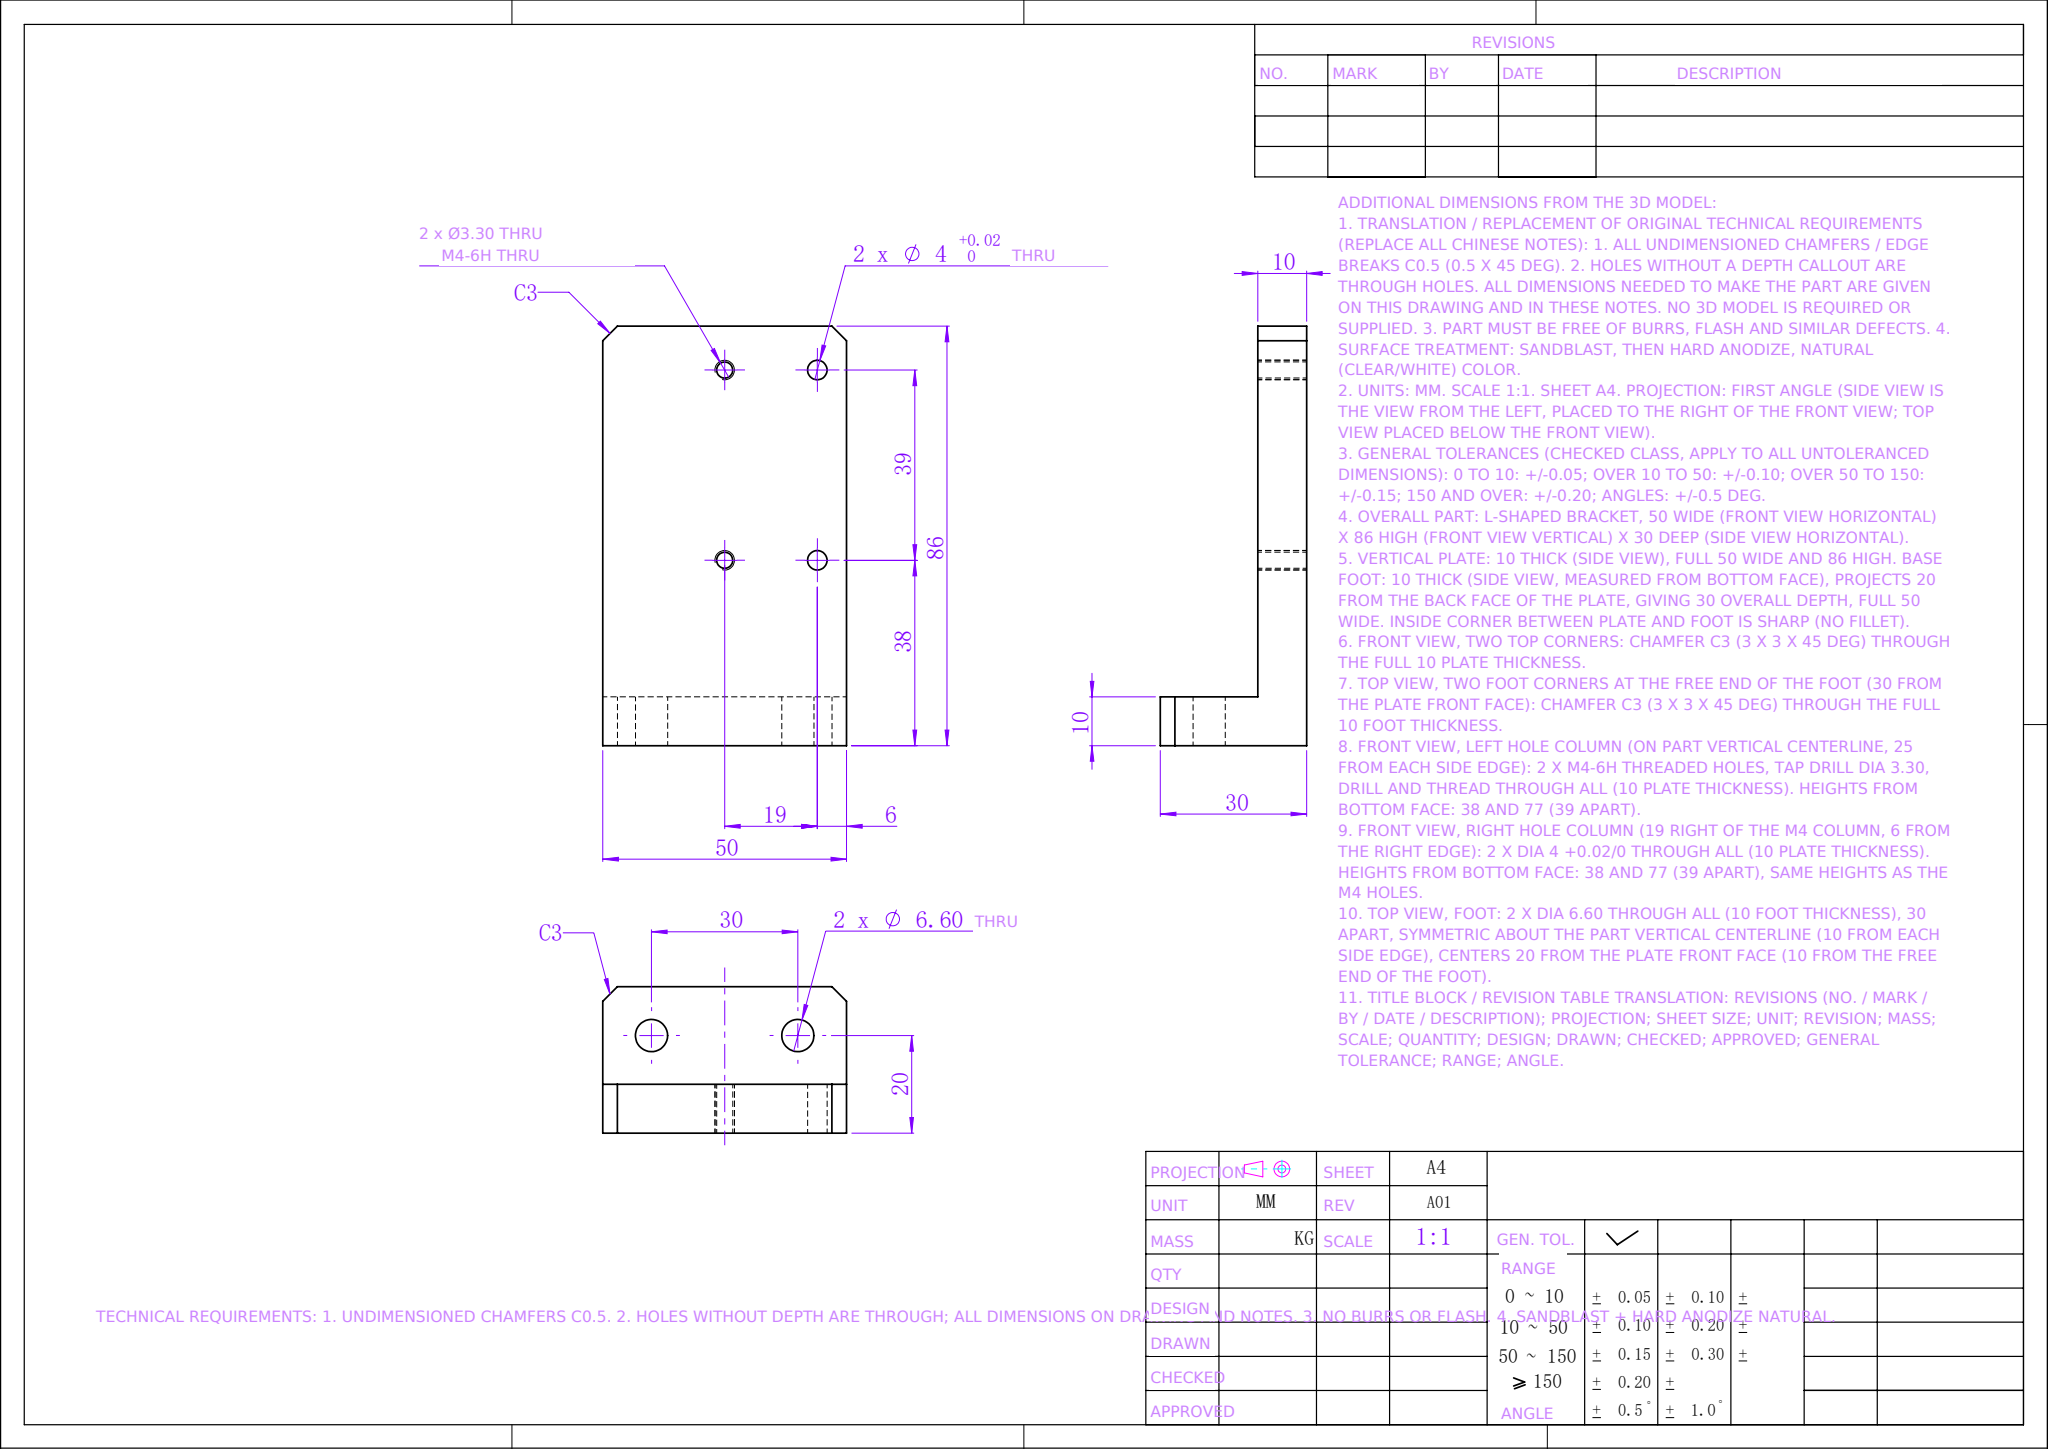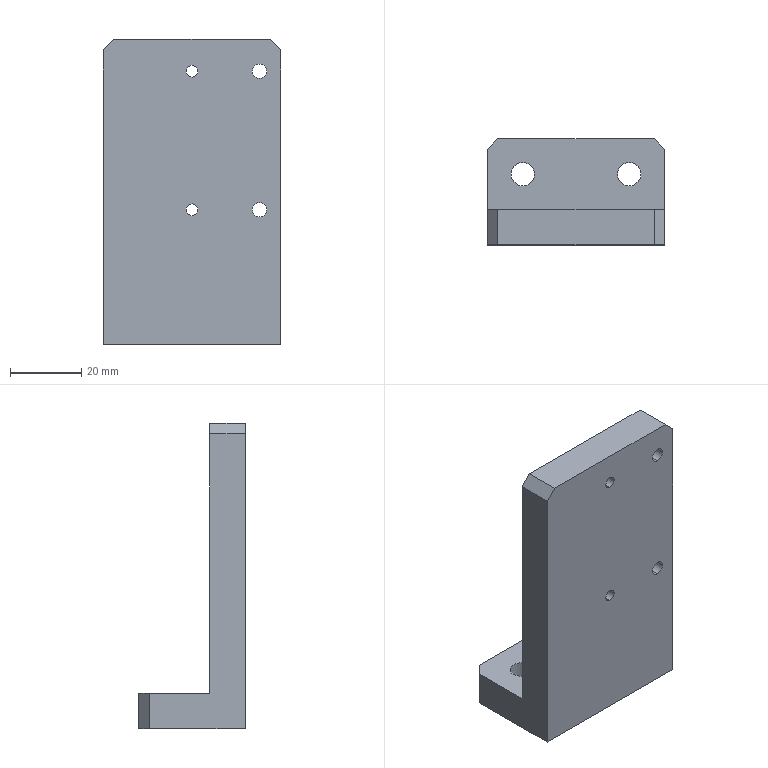Part | NX | mm | 1 solid | 24 faces | box 50 x 30 x 86 mm | volume 51713 mm3 | cylinder 12 | plane 12 | commonest cylinder face diameters 6.6 x4 4 x4 3.3 x4
STEP:
#1=COLOUR_RGB('',0.7922,0.8196,0.9333);
#2=FILL_AREA_STYLE_COLOUR('',#1);
#3=FILL_AREA_STYLE('',(#2));
#4=SURFACE_STYLE_FILL_AREA(#3);
#5=SURFACE_SIDE_STYLE('',(#4));
#6=SURFACE_STYLE_USAGE(.BOTH.,#5);
#7=PRESENTATION_STYLE_ASSIGNMENT((#6));
#8=CARTESIAN_POINT('',(-18.3,15.,-43.));
#9=VERTEX_POINT('',#8);
#10=CARTESIAN_POINT('',(-11.7,15.,-43.));
#11=VERTEX_POINT('',#10);
#12=CARTESIAN_POINT('',(-15.,15.,-43.));
#13=DIRECTION('',(0.,0.,1.));
#14=DIRECTION('',(1.,0.,0.));
#15=AXIS2_PLACEMENT_3D('',#12,#13,#14);
#16=CIRCLE('',#15,3.3);
#17=EDGE_CURVE('',#9,#11,#16,.T.);
#18=ORIENTED_EDGE('',*,*,#17,.F.);
#19=CARTESIAN_POINT('',(-18.3,15.,-33.));
#20=VERTEX_POINT('',#19);
#21=CARTESIAN_POINT('',(-18.3,15.,-33.));
#22=DIRECTION('',(0.,0.,1.));
#23=VECTOR('',#22,1000.);
#24=LINE('',#21,#23);
#25=EDGE_CURVE('',#9,#20,#24,.T.);
#26=ORIENTED_EDGE('',*,*,#25,.T.);
#27=CARTESIAN_POINT('',(-11.7,15.,-33.));
#28=VERTEX_POINT('',#27);
#29=CARTESIAN_POINT('',(-15.,15.,-33.));
#30=DIRECTION('',(0.,0.,1.));
#31=DIRECTION('',(1.,0.,0.));
#32=AXIS2_PLACEMENT_3D('',#29,#30,#31);
#33=CIRCLE('',#32,3.3);
#34=EDGE_CURVE('',#20,#28,#33,.T.);
#35=ORIENTED_EDGE('',*,*,#34,.T.);
#36=CARTESIAN_POINT('',(-11.7,15.,-33.));
#37=DIRECTION('',(0.,0.,1.));
#38=VECTOR('',#37,1000.);
#39=LINE('',#36,#38);
#40=EDGE_CURVE('',#11,#28,#39,.T.);
#41=ORIENTED_EDGE('',*,*,#40,.F.);
#42=EDGE_LOOP('',(#18,#26,#35,#41));
#43=FACE_OUTER_BOUND('',#42,.T.);
#44=CARTESIAN_POINT('',(-15.,15.,-33.));
#45=DIRECTION('',(0.,0.,1.));
#46=DIRECTION('',(1.,0.,0.));
#47=AXIS2_PLACEMENT_3D('',#44,#45,#46);
#48=CYLINDRICAL_SURFACE('',#47,3.3);
#49=ADVANCED_FACE('',(#43),#48,.F.);
#50=CARTESIAN_POINT('',(11.7,15.,-43.));
#51=VERTEX_POINT('',#50);
#52=CARTESIAN_POINT('',(18.3,15.,-43.));
#53=VERTEX_POINT('',#52);
#54=CARTESIAN_POINT('',(15.,15.,-43.));
#55=DIRECTION('',(0.,0.,1.));
#56=DIRECTION('',(1.,0.,0.));
#57=AXIS2_PLACEMENT_3D('',#54,#55,#56);
#58=CIRCLE('',#57,3.3);
#59=EDGE_CURVE('',#51,#53,#58,.T.);
#60=ORIENTED_EDGE('',*,*,#59,.F.);
#61=CARTESIAN_POINT('',(11.7,15.,-33.));
#62=VERTEX_POINT('',#61);
#63=CARTESIAN_POINT('',(11.7,15.,-33.));
#64=DIRECTION('',(0.,0.,1.));
#65=VECTOR('',#64,1000.);
#66=LINE('',#63,#65);
#67=EDGE_CURVE('',#51,#62,#66,.T.);
#68=ORIENTED_EDGE('',*,*,#67,.T.);
#69=CARTESIAN_POINT('',(18.3,15.,-33.));
#70=VERTEX_POINT('',#69);
#71=CARTESIAN_POINT('',(15.,15.,-33.));
#72=DIRECTION('',(0.,0.,1.));
#73=DIRECTION('',(1.,0.,0.));
#74=AXIS2_PLACEMENT_3D('',#71,#72,#73);
#75=CIRCLE('',#74,3.3);
#76=EDGE_CURVE('',#62,#70,#75,.T.);
#77=ORIENTED_EDGE('',*,*,#76,.T.);
#78=CARTESIAN_POINT('',(18.3,15.,-33.));
#79=DIRECTION('',(0.,0.,1.));
#80=VECTOR('',#79,1000.);
#81=LINE('',#78,#80);
#82=EDGE_CURVE('',#53,#70,#81,.T.);
#83=ORIENTED_EDGE('',*,*,#82,.F.);
#84=EDGE_LOOP('',(#60,#68,#77,#83));
#85=FACE_OUTER_BOUND('',#84,.T.);
#86=CARTESIAN_POINT('',(15.,15.,-33.));
#87=DIRECTION('',(0.,0.,1.));
#88=DIRECTION('',(1.,0.,0.));
#89=AXIS2_PLACEMENT_3D('',#86,#87,#88);
#90=CYLINDRICAL_SURFACE('',#89,3.3);
#91=ADVANCED_FACE('',(#85),#90,.F.);
#92=CARTESIAN_POINT('',(19.,-5.,32.));
#93=VERTEX_POINT('',#92);
#94=CARTESIAN_POINT('',(19.,-5.,36.));
#95=VERTEX_POINT('',#94);
#96=CARTESIAN_POINT('',(19.,-5.,34.));
#97=DIRECTION('',(0.,1.,0.));
#98=DIRECTION('',(0.,0.,1.));
#99=AXIS2_PLACEMENT_3D('',#96,#97,#98);
#100=CIRCLE('',#99,2.);
#101=EDGE_CURVE('',#93,#95,#100,.T.);
#102=ORIENTED_EDGE('',*,*,#101,.F.);
#103=CARTESIAN_POINT('',(19.,5.,32.));
#104=VERTEX_POINT('',#103);
#105=CARTESIAN_POINT('',(19.,5.,32.));
#106=DIRECTION('',(0.,1.,0.));
#107=VECTOR('',#106,1000.);
#108=LINE('',#105,#107);
#109=EDGE_CURVE('',#93,#104,#108,.T.);
#110=ORIENTED_EDGE('',*,*,#109,.T.);
#111=CARTESIAN_POINT('',(19.,5.,36.));
#112=VERTEX_POINT('',#111);
#113=CARTESIAN_POINT('',(19.,5.,34.));
#114=DIRECTION('',(0.,1.,0.));
#115=DIRECTION('',(0.,0.,1.));
#116=AXIS2_PLACEMENT_3D('',#113,#114,#115);
#117=CIRCLE('',#116,2.);
#118=EDGE_CURVE('',#104,#112,#117,.T.);
#119=ORIENTED_EDGE('',*,*,#118,.T.);
#120=CARTESIAN_POINT('',(19.,5.,36.));
#121=DIRECTION('',(0.,1.,0.));
#122=VECTOR('',#121,1000.);
#123=LINE('',#120,#122);
#124=EDGE_CURVE('',#95,#112,#123,.T.);
#125=ORIENTED_EDGE('',*,*,#124,.F.);
#126=EDGE_LOOP('',(#102,#110,#119,#125));
#127=FACE_OUTER_BOUND('',#126,.T.);
#128=CARTESIAN_POINT('',(19.,5.,34.));
#129=DIRECTION('',(0.,1.,0.));
#130=DIRECTION('',(0.,0.,1.));
#131=AXIS2_PLACEMENT_3D('',#128,#129,#130);
#132=CYLINDRICAL_SURFACE('',#131,2.);
#133=ADVANCED_FACE('',(#127),#132,.F.);
#134=CARTESIAN_POINT('',(19.,-5.,-7.));
#135=VERTEX_POINT('',#134);
#136=CARTESIAN_POINT('',(19.,-5.,-3.));
#137=VERTEX_POINT('',#136);
#138=CARTESIAN_POINT('',(19.,-5.,-5.));
#139=DIRECTION('',(0.,1.,0.));
#140=DIRECTION('',(0.,0.,1.));
#141=AXIS2_PLACEMENT_3D('',#138,#139,#140);
#142=CIRCLE('',#141,2.);
#143=EDGE_CURVE('',#135,#137,#142,.T.);
#144=ORIENTED_EDGE('',*,*,#143,.F.);
#145=CARTESIAN_POINT('',(19.,5.,-7.));
#146=VERTEX_POINT('',#145);
#147=CARTESIAN_POINT('',(19.,5.,-7.));
#148=DIRECTION('',(0.,1.,0.));
#149=VECTOR('',#148,1000.);
#150=LINE('',#147,#149);
#151=EDGE_CURVE('',#135,#146,#150,.T.);
#152=ORIENTED_EDGE('',*,*,#151,.T.);
#153=CARTESIAN_POINT('',(19.,5.,-3.));
#154=VERTEX_POINT('',#153);
#155=CARTESIAN_POINT('',(19.,5.,-5.));
#156=DIRECTION('',(0.,1.,0.));
#157=DIRECTION('',(0.,0.,1.));
#158=AXIS2_PLACEMENT_3D('',#155,#156,#157);
#159=CIRCLE('',#158,2.);
#160=EDGE_CURVE('',#146,#154,#159,.T.);
#161=ORIENTED_EDGE('',*,*,#160,.T.);
#162=CARTESIAN_POINT('',(19.,5.,-3.));
#163=DIRECTION('',(0.,1.,0.));
#164=VECTOR('',#163,1000.);
#165=LINE('',#162,#164);
#166=EDGE_CURVE('',#137,#154,#165,.T.);
#167=ORIENTED_EDGE('',*,*,#166,.F.);
#168=EDGE_LOOP('',(#144,#152,#161,#167));
#169=FACE_OUTER_BOUND('',#168,.T.);
#170=CARTESIAN_POINT('',(19.,5.,-5.));
#171=DIRECTION('',(0.,1.,0.));
#172=DIRECTION('',(0.,0.,1.));
#173=AXIS2_PLACEMENT_3D('',#170,#171,#172);
#174=CYLINDRICAL_SURFACE('',#173,2.);
#175=ADVANCED_FACE('',(#169),#174,.F.);
#176=CARTESIAN_POINT('',(-0.,5.,35.65));
#177=VERTEX_POINT('',#176);
#178=CARTESIAN_POINT('',(-0.,5.,32.35));
#179=VERTEX_POINT('',#178);
#180=CARTESIAN_POINT('',(-0.,5.,34.));
#181=DIRECTION('',(0.,-1.,0.));
#182=DIRECTION('',(0.,0.,-1.));
#183=AXIS2_PLACEMENT_3D('',#180,#181,#182);
#184=CIRCLE('',#183,1.65);
#185=EDGE_CURVE('',#177,#179,#184,.T.);
#186=ORIENTED_EDGE('',*,*,#185,.F.);
#187=CARTESIAN_POINT('',(-0.,-5.,35.65));
#188=VERTEX_POINT('',#187);
#189=CARTESIAN_POINT('',(-0.,-5.,35.65));
#190=DIRECTION('',(0.,-1.,0.));
#191=VECTOR('',#190,1000.);
#192=LINE('',#189,#191);
#193=EDGE_CURVE('',#177,#188,#192,.T.);
#194=ORIENTED_EDGE('',*,*,#193,.T.);
#195=CARTESIAN_POINT('',(-0.,-5.,32.35));
#196=VERTEX_POINT('',#195);
#197=CARTESIAN_POINT('',(-0.,-5.,34.));
#198=DIRECTION('',(0.,-1.,0.));
#199=DIRECTION('',(0.,0.,-1.));
#200=AXIS2_PLACEMENT_3D('',#197,#198,#199);
#201=CIRCLE('',#200,1.65);
#202=EDGE_CURVE('',#188,#196,#201,.T.);
#203=ORIENTED_EDGE('',*,*,#202,.T.);
#204=CARTESIAN_POINT('',(-0.,-5.,32.35));
#205=DIRECTION('',(0.,-1.,0.));
#206=VECTOR('',#205,1000.);
#207=LINE('',#204,#206);
#208=EDGE_CURVE('',#179,#196,#207,.T.);
#209=ORIENTED_EDGE('',*,*,#208,.F.);
#210=EDGE_LOOP('',(#186,#194,#203,#209));
#211=FACE_OUTER_BOUND('',#210,.T.);
#212=CARTESIAN_POINT('',(-0.,-5.,34.));
#213=DIRECTION('',(0.,-1.,0.));
#214=DIRECTION('',(0.,0.,-1.));
#215=AXIS2_PLACEMENT_3D('',#212,#213,#214);
#216=CYLINDRICAL_SURFACE('',#215,1.65);
#217=ADVANCED_FACE('',(#211),#216,.F.);
#218=CARTESIAN_POINT('',(0.,5.,-3.35));
#219=VERTEX_POINT('',#218);
#220=CARTESIAN_POINT('',(0.,5.,-6.65));
#221=VERTEX_POINT('',#220);
#222=CARTESIAN_POINT('',(0.,5.,-5.));
#223=DIRECTION('',(0.,-1.,0.));
#224=DIRECTION('',(0.,0.,-1.));
#225=AXIS2_PLACEMENT_3D('',#222,#223,#224);
#226=CIRCLE('',#225,1.65);
#227=EDGE_CURVE('',#219,#221,#226,.T.);
#228=ORIENTED_EDGE('',*,*,#227,.F.);
#229=CARTESIAN_POINT('',(0.,-5.,-3.35));
#230=VERTEX_POINT('',#229);
#231=CARTESIAN_POINT('',(0.,-5.,-3.35));
#232=DIRECTION('',(0.,-1.,0.));
#233=VECTOR('',#232,1000.);
#234=LINE('',#231,#233);
#235=EDGE_CURVE('',#219,#230,#234,.T.);
#236=ORIENTED_EDGE('',*,*,#235,.T.);
#237=CARTESIAN_POINT('',(0.,-5.,-6.65));
#238=VERTEX_POINT('',#237);
#239=CARTESIAN_POINT('',(0.,-5.,-5.));
#240=DIRECTION('',(0.,-1.,0.));
#241=DIRECTION('',(0.,0.,-1.));
#242=AXIS2_PLACEMENT_3D('',#239,#240,#241);
#243=CIRCLE('',#242,1.65);
#244=EDGE_CURVE('',#230,#238,#243,.T.);
#245=ORIENTED_EDGE('',*,*,#244,.T.);
#246=CARTESIAN_POINT('',(0.,-5.,-6.65));
#247=DIRECTION('',(0.,-1.,0.));
#248=VECTOR('',#247,1000.);
#249=LINE('',#246,#248);
#250=EDGE_CURVE('',#221,#238,#249,.T.);
#251=ORIENTED_EDGE('',*,*,#250,.F.);
#252=EDGE_LOOP('',(#228,#236,#245,#251));
#253=FACE_OUTER_BOUND('',#252,.T.);
#254=CARTESIAN_POINT('',(0.,-5.,-5.));
#255=DIRECTION('',(0.,-1.,0.));
#256=DIRECTION('',(0.,0.,-1.));
#257=AXIS2_PLACEMENT_3D('',#254,#255,#256);
#258=CYLINDRICAL_SURFACE('',#257,1.65);
#259=ADVANCED_FACE('',(#253),#258,.F.);
#260=CARTESIAN_POINT('',(19.,5.,-5.));
#261=DIRECTION('',(0.,1.,0.));
#262=DIRECTION('',(0.,0.,1.));
#263=AXIS2_PLACEMENT_3D('',#260,#261,#262);
#264=CIRCLE('',#263,2.);
#265=EDGE_CURVE('',#154,#146,#264,.T.);
#266=ORIENTED_EDGE('',*,*,#265,.F.);
#267=ORIENTED_EDGE('',*,*,#160,.F.);
#268=EDGE_LOOP('',(#266,#267));
#269=FACE_BOUND('',#268,.T.);
#270=CARTESIAN_POINT('',(-0.,5.,34.));
#271=DIRECTION('',(0.,-1.,0.));
#272=DIRECTION('',(0.,0.,-1.));
#273=AXIS2_PLACEMENT_3D('',#270,#271,#272);
#274=CIRCLE('',#273,1.65);
#275=EDGE_CURVE('',#179,#177,#274,.T.);
#276=ORIENTED_EDGE('',*,*,#275,.T.);
#277=ORIENTED_EDGE('',*,*,#185,.T.);
#278=EDGE_LOOP('',(#276,#277));
#279=FACE_BOUND('',#278,.T.);
#280=CARTESIAN_POINT('',(0.,5.,-5.));
#281=DIRECTION('',(0.,-1.,0.));
#282=DIRECTION('',(0.,0.,-1.));
#283=AXIS2_PLACEMENT_3D('',#280,#281,#282);
#284=CIRCLE('',#283,1.65);
#285=EDGE_CURVE('',#221,#219,#284,.T.);
#286=ORIENTED_EDGE('',*,*,#285,.T.);
#287=ORIENTED_EDGE('',*,*,#227,.T.);
#288=EDGE_LOOP('',(#286,#287));
#289=FACE_BOUND('',#288,.T.);
#290=CARTESIAN_POINT('',(-25.,5.,40.));
#291=VERTEX_POINT('',#290);
#292=CARTESIAN_POINT('',(-25.,5.,-33.));
#293=VERTEX_POINT('',#292);
#294=CARTESIAN_POINT('',(-25.,5.,43.));
#295=DIRECTION('',(0.,0.,-1.));
#296=VECTOR('',#295,1000.);
#297=LINE('',#294,#296);
#298=EDGE_CURVE('',#291,#293,#297,.T.);
#299=ORIENTED_EDGE('',*,*,#298,.F.);
#300=CARTESIAN_POINT('',(-22.,5.,43.));
#301=VERTEX_POINT('',#300);
#302=CARTESIAN_POINT('',(-22.,5.,43.));
#303=DIRECTION('',(0.7071,0.,0.7071));
#304=VECTOR('',#303,1000.);
#305=LINE('',#302,#304);
#306=EDGE_CURVE('',#291,#301,#305,.T.);
#307=ORIENTED_EDGE('',*,*,#306,.T.);
#308=CARTESIAN_POINT('',(22.,5.,43.));
#309=VERTEX_POINT('',#308);
#310=CARTESIAN_POINT('',(-25.,5.,43.));
#311=DIRECTION('',(-1.,0.,0.));
#312=VECTOR('',#311,1000.);
#313=LINE('',#310,#312);
#314=EDGE_CURVE('',#309,#301,#313,.T.);
#315=ORIENTED_EDGE('',*,*,#314,.F.);
#316=CARTESIAN_POINT('',(25.,5.,40.));
#317=VERTEX_POINT('',#316);
#318=CARTESIAN_POINT('',(22.,5.,43.));
#319=DIRECTION('',(0.7071,0.,-0.7071));
#320=VECTOR('',#319,1000.);
#321=LINE('',#318,#320);
#322=EDGE_CURVE('',#309,#317,#321,.T.);
#323=ORIENTED_EDGE('',*,*,#322,.T.);
#324=CARTESIAN_POINT('',(25.,5.,-33.));
#325=VERTEX_POINT('',#324);
#326=CARTESIAN_POINT('',(25.,5.,43.));
#327=DIRECTION('',(0.,0.,-1.));
#328=VECTOR('',#327,1000.);
#329=LINE('',#326,#328);
#330=EDGE_CURVE('',#317,#325,#329,.T.);
#331=ORIENTED_EDGE('',*,*,#330,.T.);
#332=CARTESIAN_POINT('',(25.,5.,-33.));
#333=DIRECTION('',(1.,0.,-0.));
#334=VECTOR('',#333,1000.);
#335=LINE('',#332,#334);
#336=EDGE_CURVE('',#293,#325,#335,.T.);
#337=ORIENTED_EDGE('',*,*,#336,.F.);
#338=EDGE_LOOP('',(#299,#307,#315,#323,#331,#337));
#339=FACE_OUTER_BOUND('',#338,.T.);
#340=CARTESIAN_POINT('',(19.,5.,34.));
#341=DIRECTION('',(0.,1.,0.));
#342=DIRECTION('',(0.,0.,1.));
#343=AXIS2_PLACEMENT_3D('',#340,#341,#342);
#344=CIRCLE('',#343,2.);
#345=EDGE_CURVE('',#112,#104,#344,.T.);
#346=ORIENTED_EDGE('',*,*,#345,.F.);
#347=ORIENTED_EDGE('',*,*,#118,.F.);
#348=EDGE_LOOP('',(#346,#347));
#349=FACE_BOUND('',#348,.T.);
#350=CARTESIAN_POINT('',(-25.,5.,43.));
#351=DIRECTION('',(0.,-1.,0.));
#352=DIRECTION('',(0.,0.,-1.));
#353=AXIS2_PLACEMENT_3D('',#350,#351,#352);
#354=PLANE('',#353);
#355=ADVANCED_FACE('',(#269,#279,#289,#339,#349),#354,.F.);
#356=CARTESIAN_POINT('',(25.,-5.,-43.));
#357=VERTEX_POINT('',#356);
#358=CARTESIAN_POINT('',(25.,22.,-43.));
#359=VERTEX_POINT('',#358);
#360=CARTESIAN_POINT('',(25.,-5.,-43.));
#361=DIRECTION('',(0.,1.,0.));
#362=VECTOR('',#361,1000.);
#363=LINE('',#360,#362);
#364=EDGE_CURVE('',#357,#359,#363,.T.);
#365=ORIENTED_EDGE('',*,*,#364,.T.);
#366=CARTESIAN_POINT('',(25.,22.,-33.));
#367=VERTEX_POINT('',#366);
#368=CARTESIAN_POINT('',(25.,22.,43.));
#369=DIRECTION('',(0.,0.,1.));
#370=VECTOR('',#369,1000.);
#371=LINE('',#368,#370);
#372=EDGE_CURVE('',#359,#367,#371,.T.);
#373=ORIENTED_EDGE('',*,*,#372,.T.);
#374=CARTESIAN_POINT('',(25.,25.,-33.));
#375=DIRECTION('',(0.,-1.,0.));
#376=VECTOR('',#375,1000.);
#377=LINE('',#374,#376);
#378=EDGE_CURVE('',#367,#325,#377,.T.);
#379=ORIENTED_EDGE('',*,*,#378,.T.);
#380=ORIENTED_EDGE('',*,*,#330,.F.);
#381=CARTESIAN_POINT('',(25.,-5.,40.));
#382=VERTEX_POINT('',#381);
#383=CARTESIAN_POINT('',(25.,-5.,40.));
#384=DIRECTION('',(0.,-1.,0.));
#385=VECTOR('',#384,1000.);
#386=LINE('',#383,#385);
#387=EDGE_CURVE('',#317,#382,#386,.T.);
#388=ORIENTED_EDGE('',*,*,#387,.T.);
#389=CARTESIAN_POINT('',(25.,-5.,43.));
#390=DIRECTION('',(0.,0.,-1.));
#391=VECTOR('',#390,1000.);
#392=LINE('',#389,#391);
#393=EDGE_CURVE('',#382,#357,#392,.T.);
#394=ORIENTED_EDGE('',*,*,#393,.T.);
#395=EDGE_LOOP('',(#365,#373,#379,#380,#388,#394));
#396=FACE_OUTER_BOUND('',#395,.T.);
#397=CARTESIAN_POINT('',(25.,-5.,43.));
#398=DIRECTION('',(-1.,0.,0.));
#399=DIRECTION('',(0.,0.,1.));
#400=AXIS2_PLACEMENT_3D('',#397,#398,#399);
#401=PLANE('',#400);
#402=ADVANCED_FACE('',(#396),#401,.F.);
#403=CARTESIAN_POINT('',(-25.,22.,-33.));
#404=VERTEX_POINT('',#403);
#405=CARTESIAN_POINT('',(-25.,25.,-33.));
#406=DIRECTION('',(0.,-1.,0.));
#407=VECTOR('',#406,1000.);
#408=LINE('',#405,#407);
#409=EDGE_CURVE('',#404,#293,#408,.T.);
#410=ORIENTED_EDGE('',*,*,#409,.F.);
#411=CARTESIAN_POINT('',(-25.,22.,-43.));
#412=VERTEX_POINT('',#411);
#413=CARTESIAN_POINT('',(-25.,22.,43.));
#414=DIRECTION('',(0.,0.,-1.));
#415=VECTOR('',#414,1000.);
#416=LINE('',#413,#415);
#417=EDGE_CURVE('',#404,#412,#416,.T.);
#418=ORIENTED_EDGE('',*,*,#417,.T.);
#419=CARTESIAN_POINT('',(-25.,-5.,-43.));
#420=VERTEX_POINT('',#419);
#421=CARTESIAN_POINT('',(-25.,-5.,-43.));
#422=DIRECTION('',(0.,-1.,0.));
#423=VECTOR('',#422,1000.);
#424=LINE('',#421,#423);
#425=EDGE_CURVE('',#412,#420,#424,.T.);
#426=ORIENTED_EDGE('',*,*,#425,.T.);
#427=CARTESIAN_POINT('',(-25.,-5.,40.));
#428=VERTEX_POINT('',#427);
#429=CARTESIAN_POINT('',(-25.,-5.,43.));
#430=DIRECTION('',(0.,0.,-1.));
#431=VECTOR('',#430,1000.);
#432=LINE('',#429,#431);
#433=EDGE_CURVE('',#428,#420,#432,.T.);
#434=ORIENTED_EDGE('',*,*,#433,.F.);
#435=CARTESIAN_POINT('',(-25.,-5.,40.));
#436=DIRECTION('',(0.,1.,0.));
#437=VECTOR('',#436,1000.);
#438=LINE('',#435,#437);
#439=EDGE_CURVE('',#428,#291,#438,.T.);
#440=ORIENTED_EDGE('',*,*,#439,.T.);
#441=ORIENTED_EDGE('',*,*,#298,.T.);
#442=EDGE_LOOP('',(#410,#418,#426,#434,#440,#441));
#443=FACE_OUTER_BOUND('',#442,.T.);
#444=CARTESIAN_POINT('',(-25.,-5.,43.));
#445=DIRECTION('',(1.,0.,0.));
#446=DIRECTION('',(0.,0.,-1.));
#447=AXIS2_PLACEMENT_3D('',#444,#445,#446);
#448=PLANE('',#447);
#449=ADVANCED_FACE('',(#443),#448,.F.);
#450=CARTESIAN_POINT('',(19.,-5.,34.));
#451=DIRECTION('',(0.,1.,0.));
#452=DIRECTION('',(0.,0.,1.));
#453=AXIS2_PLACEMENT_3D('',#450,#451,#452);
#454=CIRCLE('',#453,2.);
#455=EDGE_CURVE('',#95,#93,#454,.T.);
#456=ORIENTED_EDGE('',*,*,#455,.T.);
#457=ORIENTED_EDGE('',*,*,#101,.T.);
#458=EDGE_LOOP('',(#456,#457));
#459=FACE_BOUND('',#458,.T.);
#460=CARTESIAN_POINT('',(19.,-5.,-5.));
#461=DIRECTION('',(0.,1.,0.));
#462=DIRECTION('',(0.,0.,1.));
#463=AXIS2_PLACEMENT_3D('',#460,#461,#462);
#464=CIRCLE('',#463,2.);
#465=EDGE_CURVE('',#137,#135,#464,.T.);
#466=ORIENTED_EDGE('',*,*,#465,.T.);
#467=ORIENTED_EDGE('',*,*,#143,.T.);
#468=EDGE_LOOP('',(#466,#467));
#469=FACE_BOUND('',#468,.T.);
#470=CARTESIAN_POINT('',(-0.,-5.,34.));
#471=DIRECTION('',(0.,-1.,0.));
#472=DIRECTION('',(0.,0.,-1.));
#473=AXIS2_PLACEMENT_3D('',#470,#471,#472);
#474=CIRCLE('',#473,1.65);
#475=EDGE_CURVE('',#196,#188,#474,.T.);
#476=ORIENTED_EDGE('',*,*,#475,.F.);
#477=ORIENTED_EDGE('',*,*,#202,.F.);
#478=EDGE_LOOP('',(#476,#477));
#479=FACE_BOUND('',#478,.T.);
#480=CARTESIAN_POINT('',(0.,-5.,-5.));
#481=DIRECTION('',(0.,-1.,0.));
#482=DIRECTION('',(0.,0.,-1.));
#483=AXIS2_PLACEMENT_3D('',#480,#481,#482);
#484=CIRCLE('',#483,1.65);
#485=EDGE_CURVE('',#238,#230,#484,.T.);
#486=ORIENTED_EDGE('',*,*,#485,.F.);
#487=ORIENTED_EDGE('',*,*,#244,.F.);
#488=EDGE_LOOP('',(#486,#487));
#489=FACE_BOUND('',#488,.T.);
#490=CARTESIAN_POINT('',(-22.,-5.,43.));
#491=VERTEX_POINT('',#490);
#492=CARTESIAN_POINT('',(22.,-5.,43.));
#493=VERTEX_POINT('',#492);
#494=CARTESIAN_POINT('',(-25.,-5.,43.));
#495=DIRECTION('',(1.,0.,0.));
#496=VECTOR('',#495,1000.);
#497=LINE('',#494,#496);
#498=EDGE_CURVE('',#491,#493,#497,.T.);
#499=ORIENTED_EDGE('',*,*,#498,.F.);
#500=CARTESIAN_POINT('',(-22.,-5.,43.));
#501=DIRECTION('',(-0.7071,0.,-0.7071));
#502=VECTOR('',#501,1000.);
#503=LINE('',#500,#502);
#504=EDGE_CURVE('',#491,#428,#503,.T.);
#505=ORIENTED_EDGE('',*,*,#504,.T.);
#506=ORIENTED_EDGE('',*,*,#433,.T.);
#507=CARTESIAN_POINT('',(-25.,-5.,-43.));
#508=DIRECTION('',(1.,0.,0.));
#509=VECTOR('',#508,1000.);
#510=LINE('',#507,#509);
#511=EDGE_CURVE('',#420,#357,#510,.T.);
#512=ORIENTED_EDGE('',*,*,#511,.T.);
#513=ORIENTED_EDGE('',*,*,#393,.F.);
#514=CARTESIAN_POINT('',(22.,-5.,43.));
#515=DIRECTION('',(-0.7071,0.,0.7071));
#516=VECTOR('',#515,1000.);
#517=LINE('',#514,#516);
#518=EDGE_CURVE('',#382,#493,#517,.T.);
#519=ORIENTED_EDGE('',*,*,#518,.T.);
#520=EDGE_LOOP('',(#499,#505,#506,#512,#513,#519));
#521=FACE_OUTER_BOUND('',#520,.T.);
#522=CARTESIAN_POINT('',(-25.,-5.,43.));
#523=DIRECTION('',(0.,1.,0.));
#524=DIRECTION('',(0.,0.,1.));
#525=AXIS2_PLACEMENT_3D('',#522,#523,#524);
#526=PLANE('',#525);
#527=ADVANCED_FACE('',(#459,#469,#479,#489,#521),#526,.F.);
#528=ORIENTED_EDGE('',*,*,#314,.T.);
#529=CARTESIAN_POINT('',(-22.,0.,43.));
#530=DIRECTION('',(0.,-1.,0.));
#531=VECTOR('',#530,1000.);
#532=LINE('',#529,#531);
#533=EDGE_CURVE('',#301,#491,#532,.T.);
#534=ORIENTED_EDGE('',*,*,#533,.T.);
#535=ORIENTED_EDGE('',*,*,#498,.T.);
#536=CARTESIAN_POINT('',(22.,0.,43.));
#537=DIRECTION('',(0.,1.,0.));
#538=VECTOR('',#537,1000.);
#539=LINE('',#536,#538);
#540=EDGE_CURVE('',#493,#309,#539,.T.);
#541=ORIENTED_EDGE('',*,*,#540,.T.);
#542=EDGE_LOOP('',(#528,#534,#535,#541));
#543=FACE_OUTER_BOUND('',#542,.T.);
#544=CARTESIAN_POINT('',(0.,0.,43.));
#545=DIRECTION('',(0.,0.,-1.));
#546=DIRECTION('',(-1.,0.,0.));
#547=AXIS2_PLACEMENT_3D('',#544,#545,#546);
#548=PLANE('',#547);
#549=ADVANCED_FACE('',(#543),#548,.F.);
#550=CARTESIAN_POINT('',(-15.,15.,-43.));
#551=DIRECTION('',(0.,0.,1.));
#552=DIRECTION('',(1.,0.,0.));
#553=AXIS2_PLACEMENT_3D('',#550,#551,#552);
#554=CIRCLE('',#553,3.3);
#555=EDGE_CURVE('',#11,#9,#554,.T.);
#556=ORIENTED_EDGE('',*,*,#555,.T.);
#557=ORIENTED_EDGE('',*,*,#17,.T.);
#558=EDGE_LOOP('',(#556,#557));
#559=FACE_BOUND('',#558,.T.);
#560=CARTESIAN_POINT('',(15.,15.,-43.));
#561=DIRECTION('',(0.,0.,1.));
#562=DIRECTION('',(1.,0.,0.));
#563=AXIS2_PLACEMENT_3D('',#560,#561,#562);
#564=CIRCLE('',#563,3.3);
#565=EDGE_CURVE('',#53,#51,#564,.T.);
#566=ORIENTED_EDGE('',*,*,#565,.T.);
#567=ORIENTED_EDGE('',*,*,#59,.T.);
#568=EDGE_LOOP('',(#566,#567));
#569=FACE_BOUND('',#568,.T.);
#570=CARTESIAN_POINT('',(22.,25.,-43.));
#571=VERTEX_POINT('',#570);
#572=CARTESIAN_POINT('',(-22.,25.,-43.));
#573=VERTEX_POINT('',#572);
#574=CARTESIAN_POINT('',(25.,25.,-43.));
#575=DIRECTION('',(-1.,0.,0.));
#576=VECTOR('',#575,1000.);
#577=LINE('',#574,#576);
#578=EDGE_CURVE('',#571,#573,#577,.T.);
#579=ORIENTED_EDGE('',*,*,#578,.F.);
#580=CARTESIAN_POINT('',(23.5,23.5,-43.));
#581=DIRECTION('',(0.7071,-0.7071,0.));
#582=VECTOR('',#581,1000.);
#583=LINE('',#580,#582);
#584=EDGE_CURVE('',#571,#359,#583,.T.);
#585=ORIENTED_EDGE('',*,*,#584,.T.);
#586=ORIENTED_EDGE('',*,*,#364,.F.);
#587=ORIENTED_EDGE('',*,*,#511,.F.);
#588=ORIENTED_EDGE('',*,*,#425,.F.);
#589=CARTESIAN_POINT('',(-23.5,23.5,-43.));
#590=DIRECTION('',(0.7071,0.7071,0.));
#591=VECTOR('',#590,1000.);
#592=LINE('',#589,#591);
#593=EDGE_CURVE('',#412,#573,#592,.T.);
#594=ORIENTED_EDGE('',*,*,#593,.T.);
#595=EDGE_LOOP('',(#579,#585,#586,#587,#588,#594));
#596=FACE_OUTER_BOUND('',#595,.T.);
#597=CARTESIAN_POINT('',(0.,0.,-43.));
#598=DIRECTION('',(0.,0.,-1.));
#599=DIRECTION('',(-1.,0.,0.));
#600=AXIS2_PLACEMENT_3D('',#597,#598,#599);
#601=PLANE('',#600);
#602=ADVANCED_FACE('',(#559,#569,#596),#601,.T.);
#603=CARTESIAN_POINT('',(-15.,15.,-33.));
#604=DIRECTION('',(0.,0.,1.));
#605=DIRECTION('',(1.,0.,0.));
#606=AXIS2_PLACEMENT_3D('',#603,#604,#605);
#607=CIRCLE('',#606,3.3);
#608=EDGE_CURVE('',#28,#20,#607,.T.);
#609=ORIENTED_EDGE('',*,*,#608,.F.);
#610=ORIENTED_EDGE('',*,*,#34,.F.);
#611=EDGE_LOOP('',(#609,#610));
#612=FACE_BOUND('',#611,.T.);
#613=CARTESIAN_POINT('',(15.,15.,-33.));
#614=DIRECTION('',(0.,0.,1.));
#615=DIRECTION('',(1.,0.,0.));
#616=AXIS2_PLACEMENT_3D('',#613,#614,#615);
#617=CIRCLE('',#616,3.3);
#618=EDGE_CURVE('',#70,#62,#617,.T.);
#619=ORIENTED_EDGE('',*,*,#618,.F.);
#620=ORIENTED_EDGE('',*,*,#76,.F.);
#621=EDGE_LOOP('',(#619,#620));
#622=FACE_BOUND('',#621,.T.);
#623=ORIENTED_EDGE('',*,*,#378,.F.);
#624=CARTESIAN_POINT('',(22.,25.,-33.));
#625=VERTEX_POINT('',#624);
#626=CARTESIAN_POINT('',(22.,25.,-33.));
#627=DIRECTION('',(-0.7071,0.7071,0.));
#628=VECTOR('',#627,1000.);
#629=LINE('',#626,#628);
#630=EDGE_CURVE('',#367,#625,#629,.T.);
#631=ORIENTED_EDGE('',*,*,#630,.T.);
#632=CARTESIAN_POINT('',(-22.,25.,-33.));
#633=VERTEX_POINT('',#632);
#634=CARTESIAN_POINT('',(25.,25.,-33.));
#635=DIRECTION('',(1.,0.,-0.));
#636=VECTOR('',#635,1000.);
#637=LINE('',#634,#636);
#638=EDGE_CURVE('',#633,#625,#637,.T.);
#639=ORIENTED_EDGE('',*,*,#638,.F.);
#640=CARTESIAN_POINT('',(-22.,25.,-33.));
#641=DIRECTION('',(-0.7071,-0.7071,0.));
#642=VECTOR('',#641,1000.);
#643=LINE('',#640,#642);
#644=EDGE_CURVE('',#633,#404,#643,.T.);
#645=ORIENTED_EDGE('',*,*,#644,.T.);
#646=ORIENTED_EDGE('',*,*,#409,.T.);
#647=ORIENTED_EDGE('',*,*,#336,.T.);
#648=EDGE_LOOP('',(#623,#631,#639,#645,#646,#647));
#649=FACE_OUTER_BOUND('',#648,.T.);
#650=CARTESIAN_POINT('',(25.,25.,-33.));
#651=DIRECTION('',(-0.,0.,-1.));
#652=DIRECTION('',(-1.,0.,0.));
#653=AXIS2_PLACEMENT_3D('',#650,#651,#652);
#654=PLANE('',#653);
#655=ADVANCED_FACE('',(#612,#622,#649),#654,.F.);
#656=ORIENTED_EDGE('',*,*,#638,.T.);
#657=CARTESIAN_POINT('',(22.,25.,0.));
#658=DIRECTION('',(0.,0.,-1.));
#659=VECTOR('',#658,1000.);
#660=LINE('',#657,#659);
#661=EDGE_CURVE('',#625,#571,#660,.T.);
#662=ORIENTED_EDGE('',*,*,#661,.T.);
#663=ORIENTED_EDGE('',*,*,#578,.T.);
#664=CARTESIAN_POINT('',(-22.,25.,0.));
#665=DIRECTION('',(0.,0.,1.));
#666=VECTOR('',#665,1000.);
#667=LINE('',#664,#666);
#668=EDGE_CURVE('',#573,#633,#667,.T.);
#669=ORIENTED_EDGE('',*,*,#668,.T.);
#670=EDGE_LOOP('',(#656,#662,#663,#669));
#671=FACE_OUTER_BOUND('',#670,.T.);
#672=CARTESIAN_POINT('',(0.,25.,0.));
#673=DIRECTION('',(0.,-1.,0.));
#674=DIRECTION('',(0.,0.,-1.));
#675=AXIS2_PLACEMENT_3D('',#672,#673,#674);
#676=PLANE('',#675);
#677=ADVANCED_FACE('',(#671),#676,.F.);
#678=ORIENTED_EDGE('',*,*,#630,.F.);
#679=ORIENTED_EDGE('',*,*,#372,.F.);
#680=ORIENTED_EDGE('',*,*,#584,.F.);
#681=ORIENTED_EDGE('',*,*,#661,.F.);
#682=EDGE_LOOP('',(#678,#679,#680,#681));
#683=FACE_OUTER_BOUND('',#682,.T.);
#684=CARTESIAN_POINT('',(22.,25.,0.));
#685=DIRECTION('',(-0.7071,-0.7071,0.));
#686=DIRECTION('',(0.,0.,-1.));
#687=AXIS2_PLACEMENT_3D('',#684,#685,#686);
#688=PLANE('',#687);
#689=ADVANCED_FACE('',(#683),#688,.F.);
#690=ORIENTED_EDGE('',*,*,#593,.F.);
#691=ORIENTED_EDGE('',*,*,#417,.F.);
#692=ORIENTED_EDGE('',*,*,#644,.F.);
#693=ORIENTED_EDGE('',*,*,#668,.F.);
#694=EDGE_LOOP('',(#690,#691,#692,#693));
#695=FACE_OUTER_BOUND('',#694,.T.);
#696=CARTESIAN_POINT('',(-22.,25.,0.));
#697=DIRECTION('',(0.7071,-0.7071,0.));
#698=DIRECTION('',(0.,0.,1.));
#699=AXIS2_PLACEMENT_3D('',#696,#697,#698);
#700=PLANE('',#699);
#701=ADVANCED_FACE('',(#695),#700,.F.);
#702=ORIENTED_EDGE('',*,*,#306,.F.);
#703=ORIENTED_EDGE('',*,*,#439,.F.);
#704=ORIENTED_EDGE('',*,*,#504,.F.);
#705=ORIENTED_EDGE('',*,*,#533,.F.);
#706=EDGE_LOOP('',(#702,#703,#704,#705));
#707=FACE_OUTER_BOUND('',#706,.T.);
#708=CARTESIAN_POINT('',(-22.,0.,43.));
#709=DIRECTION('',(0.7071,0.,-0.7071));
#710=DIRECTION('',(0.,-1.,0.));
#711=AXIS2_PLACEMENT_3D('',#708,#709,#710);
#712=PLANE('',#711);
#713=ADVANCED_FACE('',(#707),#712,.F.);
#714=ORIENTED_EDGE('',*,*,#518,.F.);
#715=ORIENTED_EDGE('',*,*,#387,.F.);
#716=ORIENTED_EDGE('',*,*,#322,.F.);
#717=ORIENTED_EDGE('',*,*,#540,.F.);
#718=EDGE_LOOP('',(#714,#715,#716,#717));
#719=FACE_OUTER_BOUND('',#718,.T.);
#720=CARTESIAN_POINT('',(22.,0.,43.));
#721=DIRECTION('',(-0.7071,0.,-0.7071));
#722=DIRECTION('',(0.,1.,0.));
#723=AXIS2_PLACEMENT_3D('',#720,#721,#722);
#724=PLANE('',#723);
#725=ADVANCED_FACE('',(#719),#724,.F.);
#726=ORIENTED_EDGE('',*,*,#235,.F.);
#727=ORIENTED_EDGE('',*,*,#285,.F.);
#728=ORIENTED_EDGE('',*,*,#250,.T.);
#729=ORIENTED_EDGE('',*,*,#485,.T.);
#730=EDGE_LOOP('',(#726,#727,#728,#729));
#731=FACE_OUTER_BOUND('',#730,.T.);
#732=CARTESIAN_POINT('',(0.,-5.,-5.));
#733=DIRECTION('',(0.,-1.,0.));
#734=DIRECTION('',(0.,0.,-1.));
#735=AXIS2_PLACEMENT_3D('',#732,#733,#734);
#736=CYLINDRICAL_SURFACE('',#735,1.65);
#737=ADVANCED_FACE('',(#731),#736,.F.);
#738=ORIENTED_EDGE('',*,*,#193,.F.);
#739=ORIENTED_EDGE('',*,*,#275,.F.);
#740=ORIENTED_EDGE('',*,*,#208,.T.);
#741=ORIENTED_EDGE('',*,*,#475,.T.);
#742=EDGE_LOOP('',(#738,#739,#740,#741));
#743=FACE_OUTER_BOUND('',#742,.T.);
#744=CARTESIAN_POINT('',(-0.,-5.,34.));
#745=DIRECTION('',(0.,-1.,0.));
#746=DIRECTION('',(0.,0.,-1.));
#747=AXIS2_PLACEMENT_3D('',#744,#745,#746);
#748=CYLINDRICAL_SURFACE('',#747,1.65);
#749=ADVANCED_FACE('',(#743),#748,.F.);
#750=ORIENTED_EDGE('',*,*,#151,.F.);
#751=ORIENTED_EDGE('',*,*,#465,.F.);
#752=ORIENTED_EDGE('',*,*,#166,.T.);
#753=ORIENTED_EDGE('',*,*,#265,.T.);
#754=EDGE_LOOP('',(#750,#751,#752,#753));
#755=FACE_OUTER_BOUND('',#754,.T.);
#756=CARTESIAN_POINT('',(19.,5.,-5.));
#757=DIRECTION('',(0.,1.,0.));
#758=DIRECTION('',(0.,0.,1.));
#759=AXIS2_PLACEMENT_3D('',#756,#757,#758);
#760=CYLINDRICAL_SURFACE('',#759,2.);
#761=ADVANCED_FACE('',(#755),#760,.F.);
#762=ORIENTED_EDGE('',*,*,#109,.F.);
#763=ORIENTED_EDGE('',*,*,#455,.F.);
#764=ORIENTED_EDGE('',*,*,#124,.T.);
#765=ORIENTED_EDGE('',*,*,#345,.T.);
#766=EDGE_LOOP('',(#762,#763,#764,#765));
#767=FACE_OUTER_BOUND('',#766,.T.);
#768=CARTESIAN_POINT('',(19.,5.,34.));
#769=DIRECTION('',(0.,1.,0.));
#770=DIRECTION('',(0.,0.,1.));
#771=AXIS2_PLACEMENT_3D('',#768,#769,#770);
#772=CYLINDRICAL_SURFACE('',#771,2.);
#773=ADVANCED_FACE('',(#767),#772,.F.);
#774=ORIENTED_EDGE('',*,*,#67,.F.);
#775=ORIENTED_EDGE('',*,*,#565,.F.);
#776=ORIENTED_EDGE('',*,*,#82,.T.);
#777=ORIENTED_EDGE('',*,*,#618,.T.);
#778=EDGE_LOOP('',(#774,#775,#776,#777));
#779=FACE_OUTER_BOUND('',#778,.T.);
#780=CARTESIAN_POINT('',(15.,15.,-33.));
#781=DIRECTION('',(0.,0.,1.));
#782=DIRECTION('',(1.,0.,0.));
#783=AXIS2_PLACEMENT_3D('',#780,#781,#782);
#784=CYLINDRICAL_SURFACE('',#783,3.3);
#785=ADVANCED_FACE('',(#779),#784,.F.);
#786=ORIENTED_EDGE('',*,*,#25,.F.);
#787=ORIENTED_EDGE('',*,*,#555,.F.);
#788=ORIENTED_EDGE('',*,*,#40,.T.);
#789=ORIENTED_EDGE('',*,*,#608,.T.);
#790=EDGE_LOOP('',(#786,#787,#788,#789));
#791=FACE_OUTER_BOUND('',#790,.T.);
#792=CARTESIAN_POINT('',(-15.,15.,-33.));
#793=DIRECTION('',(0.,0.,1.));
#794=DIRECTION('',(1.,0.,0.));
#795=AXIS2_PLACEMENT_3D('',#792,#793,#794);
#796=CYLINDRICAL_SURFACE('',#795,3.3);
#797=ADVANCED_FACE('',(#791),#796,.F.);
#798=CLOSED_SHELL('',(#49,#91,#133,#175,#217,#259,#355,#402,#449,#527,#549,#602,#655,#677,#689,#701,#713,#725,#737,#749,#761,#773,#785,#797));
#799=MANIFOLD_SOLID_BREP('',#798);
#800=STYLED_ITEM('',(#7),#799);
#801=PRESENTATION_LAYER_ASSIGNMENT('','',(#800));
#802=(LENGTH_UNIT()NAMED_UNIT(*)SI_UNIT(.MILLI.,.METRE.));
#803=UNCERTAINTY_MEASURE_WITH_UNIT(LENGTH_MEASURE(0.00001),#802,'','');
#804=(NAMED_UNIT(*)PLANE_ANGLE_UNIT()SI_UNIT($,.RADIAN.));
#805=(NAMED_UNIT(*)SI_UNIT($,.STERADIAN.)SOLID_ANGLE_UNIT());
#806=(GEOMETRIC_REPRESENTATION_CONTEXT(3)GLOBAL_UNCERTAINTY_ASSIGNED_CONTEXT((#803))GLOBAL_UNIT_ASSIGNED_CONTEXT((#802,#804,#805))REPRESENTATION_CONTEXT('',''));
#807=MECHANICAL_DESIGN_GEOMETRIC_PRESENTATION_REPRESENTATION('',(#800),#806);
#808=CARTESIAN_POINT('',(0.,0.,0.));
#809=DIRECTION('',(0.,0.,1.));
#810=DIRECTION('',(1.,0.,0.));
#811=AXIS2_PLACEMENT_3D('',#808,#809,#810);
#812=(LENGTH_UNIT()NAMED_UNIT(*)SI_UNIT(.MILLI.,.METRE.));
#813=UNCERTAINTY_MEASURE_WITH_UNIT(LENGTH_MEASURE(0.00001),#812,'','');
#814=(NAMED_UNIT(*)PLANE_ANGLE_UNIT()SI_UNIT($,.RADIAN.));
#815=(NAMED_UNIT(*)SI_UNIT($,.STERADIAN.)SOLID_ANGLE_UNIT());
#816=(GEOMETRIC_REPRESENTATION_CONTEXT(3)GLOBAL_UNCERTAINTY_ASSIGNED_CONTEXT((#813))GLOBAL_UNIT_ASSIGNED_CONTEXT((#812,#814,#815))REPRESENTATION_CONTEXT('',''));
#817=ADVANCED_BREP_SHAPE_REPRESENTATION('',(#799,#811),#816);